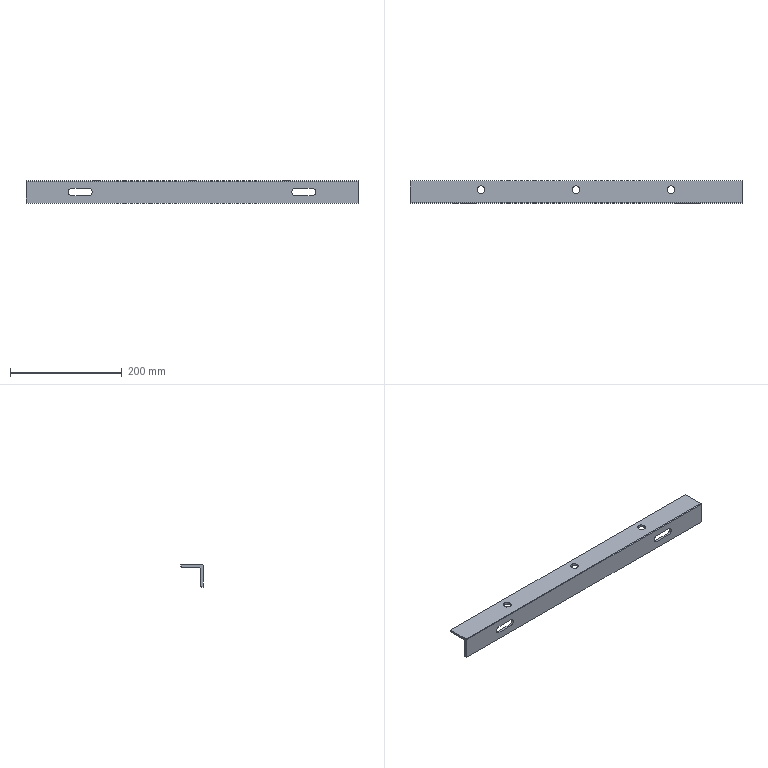Component | SolidWorks | hot-rolled equal angle gb-1 | 1 solid | 26 faces | box 594 x 40 x 40 mm | volume 177153 mm3 | cylinder 14 | plane 12 | commonest cylinder face diameters 14 x6 13 x4 2.667 x2 10 x1 2 x1
build123d program:
from build123d import *

# Parameters (mm, degrees)
BASE_DEPTH          = 594
SKETCH1_2_R         = 7
CUT_EXTRUDE1_DEPTH  = 10
LPATTERN1_COUNT     = 2
LPATTERN1_PITCH     = 170
LPATTERN1_COL_COUNT = 2
LPATTERN1_COL_PITCH = 170
CUT_EXTRUDE2_DEPTH  = 10
FILLET1_R           = 1


with BuildPart() as part:
    # Sketch1 → Base (new body)
    with BuildSketch(Plane.YZ):
        with BuildLine():
            Line((0, 40), (0, 0))
            Line((0, 0), (40, 0))
            Line((40, 0), (40, 2.667))
            ThreePointArc((40, 2.667), (39.609, 3.609), (38.667, 4))
            Line((38.667, 4), (9, 4))
            ThreePointArc((9, 4), (5.464, 5.464), (4, 9))
            Line((4, 9), (4, 38.667))
            ThreePointArc((4, 38.667), (3.609, 39.609), (2.667, 40))
            Line((2.667, 40), (0, 40))
        make_face()
    extrude(amount=BASE_DEPTH)

    # Sketch1_2 → Cut-Extrude1 (cut)
    with BuildSketch(Plane.XY.offset(4)):
        with Locations((297, 24)):
            Circle(SKETCH1_2_R)
    cut_extrude1 = extrude(amount=-CUT_EXTRUDE1_DEPTH, mode=Mode.SUBTRACT)

    # LPattern1: Cut-Extrude1 ×2
    with Locations(*[(-i * LPATTERN1_PITCH, 0, 0) for i in range(1, LPATTERN1_COUNT)]):
        add(cut_extrude1, mode=Mode.SUBTRACT)

    # LPattern1 col: Cut-Extrude1 ×2
    with Locations(*[(i * LPATTERN1_COL_PITCH, 0, 0) for i in range(1, LPATTERN1_COL_COUNT)]):
        add(cut_extrude1, mode=Mode.SUBTRACT)

    # Sketch2 → Cut-Extrude2 (cut)
    with BuildSketch(Plane(origin=(0, 4, 0), x_dir=(1, 0, 0), z_dir=(0, 1, 0))):
        with BuildLine():
            Line((82, -13.5), (112, -13.5))
            ThreePointArc((112, -13.5), (118.5, -20), (112, -26.5))
            Line((112, -26.5), (82, -26.5))
            ThreePointArc((82, -26.5), (75.5, -20), (82, -13.5))
        make_face()
        with BuildLine():
            Line((512, -13.5), (482, -13.5))
            ThreePointArc((482, -13.5), (475.5, -20), (482, -26.5))
            Line((482, -26.5), (512, -26.5))
            ThreePointArc((512, -26.5), (518.5, -20), (512, -13.5))
        make_face()
    extrude(amount=-CUT_EXTRUDE2_DEPTH, mode=Mode.SUBTRACT)

    # Fillet1
    fillet1_edges = [part.edges().sort_by_distance(p)[0] for p in [
        (297, 0, 0),
    ]]
    fillet(fillet1_edges, radius=FILLET1_R)


solid = part.part

# Placed as in the assembly
solid = solid.moved(Location((889.054, 148.5, 997), (-180, 0, 180)))
STEP:
#1=CARTESIAN_POINT('',(16.892,6.791,39.252));
#2=VERTEX_POINT('',#1);
#3=CARTESIAN_POINT('',(16.341,6.791,39.252));
#4=VERTEX_POINT('',#3);
#5=CARTESIAN_POINT('',(16.616,6.791,39.252));
#6=DIRECTION('',(0.,0.,-1.));
#7=DIRECTION('',(-1.,0.,0.));
#8=AXIS2_PLACEMENT_3D('',#5,#6,#7);
#9=CIRCLE('',#8,0.2756);
#10=EDGE_CURVE('',#2,#4,#9,.T.);
#11=ORIENTED_EDGE('',*,*,#10,.F.);
#12=CARTESIAN_POINT('',(16.892,6.791,39.094));
#13=VERTEX_POINT('',#12);
#14=CARTESIAN_POINT('',(16.892,6.791,39.488));
#15=DIRECTION('',(0.,0.,-1.));
#16=VECTOR('',#15,39.37);
#17=LINE('',#14,#16);
#18=EDGE_CURVE('',#2,#13,#17,.T.);
#19=ORIENTED_EDGE('',*,*,#18,.T.);
#20=CARTESIAN_POINT('',(16.341,6.791,39.094));
#21=VERTEX_POINT('',#20);
#22=CARTESIAN_POINT('',(16.616,6.791,39.094));
#23=DIRECTION('',(0.,0.,-1.));
#24=DIRECTION('',(-1.,0.,0.));
#25=AXIS2_PLACEMENT_3D('',#22,#23,#24);
#26=CIRCLE('',#25,0.2756);
#27=EDGE_CURVE('',#13,#21,#26,.T.);
#28=ORIENTED_EDGE('',*,*,#27,.T.);
#29=CARTESIAN_POINT('',(16.341,6.791,39.488));
#30=DIRECTION('',(0.,0.,-1.));
#31=VECTOR('',#30,39.37);
#32=LINE('',#29,#31);
#33=EDGE_CURVE('',#4,#21,#32,.T.);
#34=ORIENTED_EDGE('',*,*,#33,.F.);
#35=EDGE_LOOP('',(#11,#19,#28,#34));
#36=FACE_OUTER_BOUND('',#35,.T.);
#37=CARTESIAN_POINT('',(16.616,6.791,39.488));
#38=DIRECTION('',(0.,0.,-1.));
#39=DIRECTION('',(-1.,0.,0.));
#40=AXIS2_PLACEMENT_3D('',#37,#38,#39);
#41=CYLINDRICAL_SURFACE('',#40,0.2756);
#42=ADVANCED_FACE('',(#36),#41,.F.);
#43=CARTESIAN_POINT('',(30.278,6.791,39.252));
#44=VERTEX_POINT('',#43);
#45=CARTESIAN_POINT('',(29.727,6.791,39.252));
#46=VERTEX_POINT('',#45);
#47=CARTESIAN_POINT('',(30.002,6.791,39.252));
#48=DIRECTION('',(0.,0.,-1.));
#49=DIRECTION('',(-1.,0.,0.));
#50=AXIS2_PLACEMENT_3D('',#47,#48,#49);
#51=CIRCLE('',#50,0.2756);
#52=EDGE_CURVE('',#44,#46,#51,.T.);
#53=ORIENTED_EDGE('',*,*,#52,.F.);
#54=CARTESIAN_POINT('',(30.278,6.791,39.094));
#55=VERTEX_POINT('',#54);
#56=CARTESIAN_POINT('',(30.278,6.791,39.488));
#57=DIRECTION('',(0.,0.,-1.));
#58=VECTOR('',#57,39.37);
#59=LINE('',#56,#58);
#60=EDGE_CURVE('',#44,#55,#59,.T.);
#61=ORIENTED_EDGE('',*,*,#60,.T.);
#62=CARTESIAN_POINT('',(29.727,6.791,39.094));
#63=VERTEX_POINT('',#62);
#64=CARTESIAN_POINT('',(30.002,6.791,39.094));
#65=DIRECTION('',(0.,0.,-1.));
#66=DIRECTION('',(-1.,0.,0.));
#67=AXIS2_PLACEMENT_3D('',#64,#65,#66);
#68=CIRCLE('',#67,0.2756);
#69=EDGE_CURVE('',#55,#63,#68,.T.);
#70=ORIENTED_EDGE('',*,*,#69,.T.);
#71=CARTESIAN_POINT('',(29.727,6.791,39.488));
#72=DIRECTION('',(0.,0.,-1.));
#73=VECTOR('',#72,39.37);
#74=LINE('',#71,#73);
#75=EDGE_CURVE('',#46,#63,#74,.T.);
#76=ORIENTED_EDGE('',*,*,#75,.F.);
#77=EDGE_LOOP('',(#53,#61,#70,#76));
#78=FACE_OUTER_BOUND('',#77,.T.);
#79=CARTESIAN_POINT('',(30.002,6.791,39.488));
#80=DIRECTION('',(0.,0.,-1.));
#81=DIRECTION('',(-1.,0.,0.));
#82=AXIS2_PLACEMENT_3D('',#79,#80,#81);
#83=CYLINDRICAL_SURFACE('',#82,0.2756);
#84=ADVANCED_FACE('',(#78),#83,.F.);
#85=CARTESIAN_POINT('',(23.585,6.791,39.252));
#86=VERTEX_POINT('',#85);
#87=CARTESIAN_POINT('',(23.034,6.791,39.252));
#88=VERTEX_POINT('',#87);
#89=CARTESIAN_POINT('',(23.309,6.791,39.252));
#90=DIRECTION('',(0.,0.,-1.));
#91=DIRECTION('',(-1.,0.,0.));
#92=AXIS2_PLACEMENT_3D('',#89,#90,#91);
#93=CIRCLE('',#92,0.2756);
#94=EDGE_CURVE('',#86,#88,#93,.T.);
#95=ORIENTED_EDGE('',*,*,#94,.F.);
#96=CARTESIAN_POINT('',(23.585,6.791,39.094));
#97=VERTEX_POINT('',#96);
#98=CARTESIAN_POINT('',(23.585,6.791,39.488));
#99=DIRECTION('',(0.,0.,-1.));
#100=VECTOR('',#99,39.37);
#101=LINE('',#98,#100);
#102=EDGE_CURVE('',#86,#97,#101,.T.);
#103=ORIENTED_EDGE('',*,*,#102,.T.);
#104=CARTESIAN_POINT('',(23.034,6.791,39.094));
#105=VERTEX_POINT('',#104);
#106=CARTESIAN_POINT('',(23.309,6.791,39.094));
#107=DIRECTION('',(0.,0.,-1.));
#108=DIRECTION('',(-1.,0.,0.));
#109=AXIS2_PLACEMENT_3D('',#106,#107,#108);
#110=CIRCLE('',#109,0.2756);
#111=EDGE_CURVE('',#97,#105,#110,.T.);
#112=ORIENTED_EDGE('',*,*,#111,.T.);
#113=CARTESIAN_POINT('',(23.034,6.791,39.488));
#114=DIRECTION('',(0.,0.,-1.));
#115=VECTOR('',#114,39.37);
#116=LINE('',#113,#115);
#117=EDGE_CURVE('',#88,#105,#116,.T.);
#118=ORIENTED_EDGE('',*,*,#117,.F.);
#119=EDGE_LOOP('',(#95,#103,#112,#118));
#120=FACE_OUTER_BOUND('',#119,.T.);
#121=CARTESIAN_POINT('',(23.309,6.791,39.488));
#122=DIRECTION('',(0.,0.,-1.));
#123=DIRECTION('',(-1.,0.,0.));
#124=AXIS2_PLACEMENT_3D('',#121,#122,#123);
#125=CYLINDRICAL_SURFACE('',#124,0.2756);
#126=ADVANCED_FACE('',(#120),#125,.F.);
#127=CARTESIAN_POINT('',(35.002,5.951,37.677));
#128=VERTEX_POINT('',#127);
#129=CARTESIAN_POINT('',(35.002,5.846,37.677));
#130=VERTEX_POINT('',#129);
#131=CARTESIAN_POINT('',(35.002,5.846,37.677));
#132=DIRECTION('',(0.,-1.,0.));
#133=VECTOR('',#132,39.37);
#134=LINE('',#131,#133);
#135=EDGE_CURVE('',#128,#130,#134,.T.);
#136=ORIENTED_EDGE('',*,*,#135,.T.);
#137=CARTESIAN_POINT('',(11.616,5.846,37.677));
#138=VERTEX_POINT('',#137);
#139=CARTESIAN_POINT('',(11.616,5.846,37.677));
#140=DIRECTION('',(1.,0.,0.));
#141=VECTOR('',#140,39.37);
#142=LINE('',#139,#141);
#143=EDGE_CURVE('',#138,#130,#142,.T.);
#144=ORIENTED_EDGE('',*,*,#143,.F.);
#145=CARTESIAN_POINT('',(11.616,5.951,37.677));
#146=VERTEX_POINT('',#145);
#147=CARTESIAN_POINT('',(11.616,5.846,37.677));
#148=DIRECTION('',(0.,-1.,0.));
#149=VECTOR('',#148,39.37);
#150=LINE('',#147,#149);
#151=EDGE_CURVE('',#146,#138,#150,.T.);
#152=ORIENTED_EDGE('',*,*,#151,.F.);
#153=CARTESIAN_POINT('',(11.616,5.951,37.677));
#154=DIRECTION('',(1.,0.,0.));
#155=VECTOR('',#154,39.37);
#156=LINE('',#153,#155);
#157=EDGE_CURVE('',#146,#128,#156,.T.);
#158=ORIENTED_EDGE('',*,*,#157,.T.);
#159=EDGE_LOOP('',(#136,#144,#152,#158));
#160=FACE_OUTER_BOUND('',#159,.T.);
#161=CARTESIAN_POINT('',(11.616,5.846,37.677));
#162=DIRECTION('',(0.,0.,1.));
#163=DIRECTION('',(1.,0.,0.));
#164=AXIS2_PLACEMENT_3D('',#161,#162,#163);
#165=PLANE('',#164);
#166=ADVANCED_FACE('',(#160),#165,.F.);
#167=CARTESIAN_POINT('',(16.026,5.846,38.209));
#168=VERTEX_POINT('',#167);
#169=CARTESIAN_POINT('',(14.845,5.846,38.209));
#170=VERTEX_POINT('',#169);
#171=CARTESIAN_POINT('',(11.616,5.846,38.209));
#172=DIRECTION('',(-1.,-0.,-0.));
#173=VECTOR('',#172,39.37);
#174=LINE('',#171,#173);
#175=EDGE_CURVE('',#168,#170,#174,.T.);
#176=ORIENTED_EDGE('',*,*,#175,.T.);
#177=CARTESIAN_POINT('',(14.845,5.846,38.72));
#178=VERTEX_POINT('',#177);
#179=CARTESIAN_POINT('',(14.845,5.846,38.465));
#180=DIRECTION('',(-0.,1.,-0.));
#181=DIRECTION('',(0.,0.,-1.));
#182=AXIS2_PLACEMENT_3D('',#179,#180,#181);
#183=CIRCLE('',#182,0.2559);
#184=EDGE_CURVE('',#170,#178,#183,.T.);
#185=ORIENTED_EDGE('',*,*,#184,.T.);
#186=CARTESIAN_POINT('',(16.026,5.846,38.72));
#187=VERTEX_POINT('',#186);
#188=CARTESIAN_POINT('',(11.616,5.846,38.72));
#189=DIRECTION('',(1.,0.,0.));
#190=VECTOR('',#189,39.37);
#191=LINE('',#188,#190);
#192=EDGE_CURVE('',#178,#187,#191,.T.);
#193=ORIENTED_EDGE('',*,*,#192,.T.);
#194=CARTESIAN_POINT('',(16.026,5.846,38.465));
#195=DIRECTION('',(-0.,1.,-0.));
#196=DIRECTION('',(0.,0.,-1.));
#197=AXIS2_PLACEMENT_3D('',#194,#195,#196);
#198=CIRCLE('',#197,0.2559);
#199=EDGE_CURVE('',#187,#168,#198,.T.);
#200=ORIENTED_EDGE('',*,*,#199,.T.);
#201=EDGE_LOOP('',(#176,#185,#193,#200));
#202=FACE_BOUND('',#201,.T.);
#203=CARTESIAN_POINT('',(30.593,5.846,38.72));
#204=VERTEX_POINT('',#203);
#205=CARTESIAN_POINT('',(31.774,5.846,38.72));
#206=VERTEX_POINT('',#205);
#207=CARTESIAN_POINT('',(11.616,5.846,38.72));
#208=DIRECTION('',(1.,0.,-0.));
#209=VECTOR('',#208,39.37);
#210=LINE('',#207,#209);
#211=EDGE_CURVE('',#204,#206,#210,.T.);
#212=ORIENTED_EDGE('',*,*,#211,.T.);
#213=CARTESIAN_POINT('',(31.774,5.846,38.209));
#214=VERTEX_POINT('',#213);
#215=CARTESIAN_POINT('',(31.774,5.846,38.465));
#216=DIRECTION('',(-0.,1.,-0.));
#217=DIRECTION('',(0.,0.,-1.));
#218=AXIS2_PLACEMENT_3D('',#215,#216,#217);
#219=CIRCLE('',#218,0.2559);
#220=EDGE_CURVE('',#206,#214,#219,.T.);
#221=ORIENTED_EDGE('',*,*,#220,.T.);
#222=CARTESIAN_POINT('',(30.593,5.846,38.209));
#223=VERTEX_POINT('',#222);
#224=CARTESIAN_POINT('',(11.616,5.846,38.209));
#225=DIRECTION('',(-1.,-0.,0.));
#226=VECTOR('',#225,39.37);
#227=LINE('',#224,#226);
#228=EDGE_CURVE('',#214,#223,#227,.T.);
#229=ORIENTED_EDGE('',*,*,#228,.T.);
#230=CARTESIAN_POINT('',(30.593,5.846,38.465));
#231=DIRECTION('',(-0.,1.,-0.));
#232=DIRECTION('',(0.,0.,-1.));
#233=AXIS2_PLACEMENT_3D('',#230,#231,#232);
#234=CIRCLE('',#233,0.2559);
#235=EDGE_CURVE('',#223,#204,#234,.T.);
#236=ORIENTED_EDGE('',*,*,#235,.T.);
#237=EDGE_LOOP('',(#212,#221,#229,#236));
#238=FACE_BOUND('',#237,.T.);
#239=CARTESIAN_POINT('',(35.002,5.846,39.213));
#240=VERTEX_POINT('',#239);
#241=CARTESIAN_POINT('',(35.002,5.846,37.677));
#242=DIRECTION('',(-0.,0.,1.));
#243=VECTOR('',#242,39.37);
#244=LINE('',#241,#243);
#245=EDGE_CURVE('',#130,#240,#244,.T.);
#246=ORIENTED_EDGE('',*,*,#245,.T.);
#247=CARTESIAN_POINT('',(11.616,5.846,39.213));
#248=VERTEX_POINT('',#247);
#249=CARTESIAN_POINT('',(11.616,5.846,39.213));
#250=DIRECTION('',(-1.,-0.,0.));
#251=VECTOR('',#250,39.37);
#252=LINE('',#249,#251);
#253=EDGE_CURVE('',#240,#248,#252,.T.);
#254=ORIENTED_EDGE('',*,*,#253,.T.);
#255=CARTESIAN_POINT('',(11.616,5.846,37.677));
#256=DIRECTION('',(-0.,0.,1.));
#257=VECTOR('',#256,39.37);
#258=LINE('',#255,#257);
#259=EDGE_CURVE('',#138,#248,#258,.T.);
#260=ORIENTED_EDGE('',*,*,#259,.F.);
#261=ORIENTED_EDGE('',*,*,#143,.T.);
#262=EDGE_LOOP('',(#246,#254,#260,#261));
#263=FACE_OUTER_BOUND('',#262,.T.);
#264=CARTESIAN_POINT('',(11.616,5.846,37.677));
#265=DIRECTION('',(-0.,1.,-0.));
#266=DIRECTION('',(0.,-0.,-1.));
#267=AXIS2_PLACEMENT_3D('',#264,#265,#266);
#268=PLANE('',#267);
#269=ADVANCED_FACE('',(#202,#238,#263),#268,.F.);
#270=CARTESIAN_POINT('',(30.002,6.791,39.252));
#271=DIRECTION('',(0.,0.,-1.));
#272=DIRECTION('',(-1.,0.,0.));
#273=AXIS2_PLACEMENT_3D('',#270,#271,#272);
#274=CIRCLE('',#273,0.2756);
#275=EDGE_CURVE('',#46,#44,#274,.T.);
#276=ORIENTED_EDGE('',*,*,#275,.T.);
#277=ORIENTED_EDGE('',*,*,#52,.T.);
#278=EDGE_LOOP('',(#276,#277));
#279=FACE_BOUND('',#278,.T.);
#280=CARTESIAN_POINT('',(23.309,6.791,39.252));
#281=DIRECTION('',(0.,0.,-1.));
#282=DIRECTION('',(-1.,0.,0.));
#283=AXIS2_PLACEMENT_3D('',#280,#281,#282);
#284=CIRCLE('',#283,0.2756);
#285=EDGE_CURVE('',#88,#86,#284,.T.);
#286=ORIENTED_EDGE('',*,*,#285,.T.);
#287=ORIENTED_EDGE('',*,*,#94,.T.);
#288=EDGE_LOOP('',(#286,#287));
#289=FACE_BOUND('',#288,.T.);
#290=CARTESIAN_POINT('',(11.616,5.886,39.252));
#291=VERTEX_POINT('',#290);
#292=CARTESIAN_POINT('',(11.616,7.421,39.252));
#293=VERTEX_POINT('',#292);
#294=CARTESIAN_POINT('',(11.616,5.846,39.252));
#295=DIRECTION('',(-0.,1.,0.));
#296=VECTOR('',#295,39.37);
#297=LINE('',#294,#296);
#298=EDGE_CURVE('',#291,#293,#297,.T.);
#299=ORIENTED_EDGE('',*,*,#298,.F.);
#300=CARTESIAN_POINT('',(35.002,5.886,39.252));
#301=VERTEX_POINT('',#300);
#302=CARTESIAN_POINT('',(11.616,5.886,39.252));
#303=DIRECTION('',(1.,0.,0.));
#304=VECTOR('',#303,39.37);
#305=LINE('',#302,#304);
#306=EDGE_CURVE('',#291,#301,#305,.T.);
#307=ORIENTED_EDGE('',*,*,#306,.T.);
#308=CARTESIAN_POINT('',(35.002,7.421,39.252));
#309=VERTEX_POINT('',#308);
#310=CARTESIAN_POINT('',(35.002,5.846,39.252));
#311=DIRECTION('',(-0.,1.,0.));
#312=VECTOR('',#311,39.37);
#313=LINE('',#310,#312);
#314=EDGE_CURVE('',#301,#309,#313,.T.);
#315=ORIENTED_EDGE('',*,*,#314,.T.);
#316=CARTESIAN_POINT('',(11.616,7.421,39.252));
#317=DIRECTION('',(1.,0.,0.));
#318=VECTOR('',#317,39.37);
#319=LINE('',#316,#318);
#320=EDGE_CURVE('',#293,#309,#319,.T.);
#321=ORIENTED_EDGE('',*,*,#320,.F.);
#322=EDGE_LOOP('',(#299,#307,#315,#321));
#323=FACE_OUTER_BOUND('',#322,.T.);
#324=CARTESIAN_POINT('',(16.616,6.791,39.252));
#325=DIRECTION('',(0.,0.,-1.));
#326=DIRECTION('',(-1.,0.,0.));
#327=AXIS2_PLACEMENT_3D('',#324,#325,#326);
#328=CIRCLE('',#327,0.2756);
#329=EDGE_CURVE('',#4,#2,#328,.T.);
#330=ORIENTED_EDGE('',*,*,#329,.T.);
#331=ORIENTED_EDGE('',*,*,#10,.T.);
#332=EDGE_LOOP('',(#330,#331));
#333=FACE_BOUND('',#332,.T.);
#334=CARTESIAN_POINT('',(11.616,5.846,39.252));
#335=DIRECTION('',(0.,0.,-1.));
#336=DIRECTION('',(-1.,-0.,0.));
#337=AXIS2_PLACEMENT_3D('',#334,#335,#336);
#338=PLANE('',#337);
#339=ADVANCED_FACE('',(#279,#289,#323,#333),#338,.F.);
#340=CARTESIAN_POINT('',(35.002,7.421,39.147));
#341=VERTEX_POINT('',#340);
#342=CARTESIAN_POINT('',(35.002,7.421,39.252));
#343=DIRECTION('',(0.,0.,-1.));
#344=VECTOR('',#343,39.37);
#345=LINE('',#342,#344);
#346=EDGE_CURVE('',#309,#341,#345,.T.);
#347=ORIENTED_EDGE('',*,*,#346,.T.);
#348=CARTESIAN_POINT('',(11.616,7.421,39.147));
#349=VERTEX_POINT('',#348);
#350=CARTESIAN_POINT('',(11.616,7.421,39.147));
#351=DIRECTION('',(1.,0.,0.));
#352=VECTOR('',#351,39.37);
#353=LINE('',#350,#352);
#354=EDGE_CURVE('',#349,#341,#353,.T.);
#355=ORIENTED_EDGE('',*,*,#354,.F.);
#356=CARTESIAN_POINT('',(11.616,7.421,39.252));
#357=DIRECTION('',(0.,0.,-1.));
#358=VECTOR('',#357,39.37);
#359=LINE('',#356,#358);
#360=EDGE_CURVE('',#293,#349,#359,.T.);
#361=ORIENTED_EDGE('',*,*,#360,.F.);
#362=ORIENTED_EDGE('',*,*,#320,.T.);
#363=EDGE_LOOP('',(#347,#355,#361,#362));
#364=FACE_OUTER_BOUND('',#363,.T.);
#365=CARTESIAN_POINT('',(11.616,7.421,39.252));
#366=DIRECTION('',(0.,-1.,0.));
#367=DIRECTION('',(0.,0.,1.));
#368=AXIS2_PLACEMENT_3D('',#365,#366,#367);
#369=PLANE('',#368);
#370=ADVANCED_FACE('',(#364),#369,.F.);
#371=CARTESIAN_POINT('',(35.002,7.369,39.094));
#372=VERTEX_POINT('',#371);
#373=CARTESIAN_POINT('',(35.002,7.369,39.147));
#374=DIRECTION('',(-1.,-0.,0.));
#375=DIRECTION('',(0.,0.,1.));
#376=AXIS2_PLACEMENT_3D('',#373,#374,#375);
#377=CIRCLE('',#376,0.05249);
#378=EDGE_CURVE('',#341,#372,#377,.T.);
#379=ORIENTED_EDGE('',*,*,#378,.T.);
#380=CARTESIAN_POINT('',(11.616,7.369,39.094));
#381=VERTEX_POINT('',#380);
#382=CARTESIAN_POINT('',(11.616,7.369,39.094));
#383=DIRECTION('',(1.,0.,0.));
#384=VECTOR('',#383,39.37);
#385=LINE('',#382,#384);
#386=EDGE_CURVE('',#381,#372,#385,.T.);
#387=ORIENTED_EDGE('',*,*,#386,.F.);
#388=CARTESIAN_POINT('',(11.616,7.369,39.147));
#389=DIRECTION('',(-1.,-0.,0.));
#390=DIRECTION('',(0.,0.,1.));
#391=AXIS2_PLACEMENT_3D('',#388,#389,#390);
#392=CIRCLE('',#391,0.05249);
#393=EDGE_CURVE('',#349,#381,#392,.T.);
#394=ORIENTED_EDGE('',*,*,#393,.F.);
#395=ORIENTED_EDGE('',*,*,#354,.T.);
#396=EDGE_LOOP('',(#379,#387,#394,#395));
#397=FACE_OUTER_BOUND('',#396,.T.);
#398=CARTESIAN_POINT('',(11.616,7.369,39.147));
#399=DIRECTION('',(1.,0.,0.));
#400=DIRECTION('',(0.,0.,-1.));
#401=AXIS2_PLACEMENT_3D('',#398,#399,#400);
#402=CYLINDRICAL_SURFACE('',#401,0.05249);
#403=ADVANCED_FACE('',(#397),#402,.T.);
#404=CARTESIAN_POINT('',(30.002,6.791,39.094));
#405=DIRECTION('',(0.,0.,-1.));
#406=DIRECTION('',(-1.,0.,0.));
#407=AXIS2_PLACEMENT_3D('',#404,#405,#406);
#408=CIRCLE('',#407,0.2756);
#409=EDGE_CURVE('',#63,#55,#408,.T.);
#410=ORIENTED_EDGE('',*,*,#409,.F.);
#411=ORIENTED_EDGE('',*,*,#69,.F.);
#412=EDGE_LOOP('',(#410,#411));
#413=FACE_BOUND('',#412,.T.);
#414=CARTESIAN_POINT('',(23.309,6.791,39.094));
#415=DIRECTION('',(0.,0.,-1.));
#416=DIRECTION('',(-1.,0.,0.));
#417=AXIS2_PLACEMENT_3D('',#414,#415,#416);
#418=CIRCLE('',#417,0.2756);
#419=EDGE_CURVE('',#105,#97,#418,.T.);
#420=ORIENTED_EDGE('',*,*,#419,.F.);
#421=ORIENTED_EDGE('',*,*,#111,.F.);
#422=EDGE_LOOP('',(#420,#421));
#423=FACE_BOUND('',#422,.T.);
#424=CARTESIAN_POINT('',(35.002,6.201,39.094));
#425=VERTEX_POINT('',#424);
#426=CARTESIAN_POINT('',(35.002,6.201,39.094));
#427=DIRECTION('',(0.,-1.,0.));
#428=VECTOR('',#427,39.37);
#429=LINE('',#426,#428);
#430=EDGE_CURVE('',#372,#425,#429,.T.);
#431=ORIENTED_EDGE('',*,*,#430,.T.);
#432=CARTESIAN_POINT('',(11.616,6.201,39.094));
#433=VERTEX_POINT('',#432);
#434=CARTESIAN_POINT('',(11.616,6.201,39.094));
#435=DIRECTION('',(1.,0.,0.));
#436=VECTOR('',#435,39.37);
#437=LINE('',#434,#436);
#438=EDGE_CURVE('',#433,#425,#437,.T.);
#439=ORIENTED_EDGE('',*,*,#438,.F.);
#440=CARTESIAN_POINT('',(11.616,6.201,39.094));
#441=DIRECTION('',(0.,-1.,0.));
#442=VECTOR('',#441,39.37);
#443=LINE('',#440,#442);
#444=EDGE_CURVE('',#381,#433,#443,.T.);
#445=ORIENTED_EDGE('',*,*,#444,.F.);
#446=ORIENTED_EDGE('',*,*,#386,.T.);
#447=EDGE_LOOP('',(#431,#439,#445,#446));
#448=FACE_OUTER_BOUND('',#447,.T.);
#449=CARTESIAN_POINT('',(16.616,6.791,39.094));
#450=DIRECTION('',(0.,0.,-1.));
#451=DIRECTION('',(-1.,0.,0.));
#452=AXIS2_PLACEMENT_3D('',#449,#450,#451);
#453=CIRCLE('',#452,0.2756);
#454=EDGE_CURVE('',#21,#13,#453,.T.);
#455=ORIENTED_EDGE('',*,*,#454,.F.);
#456=ORIENTED_EDGE('',*,*,#27,.F.);
#457=EDGE_LOOP('',(#455,#456));
#458=FACE_BOUND('',#457,.T.);
#459=CARTESIAN_POINT('',(11.616,6.201,39.094));
#460=DIRECTION('',(-0.,0.,1.));
#461=DIRECTION('',(-0.,1.,-0.));
#462=AXIS2_PLACEMENT_3D('',#459,#460,#461);
#463=PLANE('',#462);
#464=ADVANCED_FACE('',(#413,#423,#448,#458),#463,.F.);
#465=CARTESIAN_POINT('',(35.002,6.004,38.898));
#466=VERTEX_POINT('',#465);
#467=CARTESIAN_POINT('',(35.002,6.201,38.898));
#468=DIRECTION('',(1.,0.,0.));
#469=DIRECTION('',(0.,0.,1.));
#470=AXIS2_PLACEMENT_3D('',#467,#468,#469);
#471=CIRCLE('',#470,0.1969);
#472=EDGE_CURVE('',#425,#466,#471,.T.);
#473=ORIENTED_EDGE('',*,*,#472,.T.);
#474=CARTESIAN_POINT('',(11.616,6.004,38.898));
#475=VERTEX_POINT('',#474);
#476=CARTESIAN_POINT('',(11.616,6.004,38.898));
#477=DIRECTION('',(1.,0.,0.));
#478=VECTOR('',#477,39.37);
#479=LINE('',#476,#478);
#480=EDGE_CURVE('',#475,#466,#479,.T.);
#481=ORIENTED_EDGE('',*,*,#480,.F.);
#482=CARTESIAN_POINT('',(11.616,6.201,38.898));
#483=DIRECTION('',(1.,0.,0.));
#484=DIRECTION('',(0.,0.,1.));
#485=AXIS2_PLACEMENT_3D('',#482,#483,#484);
#486=CIRCLE('',#485,0.1969);
#487=EDGE_CURVE('',#433,#475,#486,.T.);
#488=ORIENTED_EDGE('',*,*,#487,.F.);
#489=ORIENTED_EDGE('',*,*,#438,.T.);
#490=EDGE_LOOP('',(#473,#481,#488,#489));
#491=FACE_OUTER_BOUND('',#490,.T.);
#492=CARTESIAN_POINT('',(11.616,6.201,38.898));
#493=DIRECTION('',(1.,0.,0.));
#494=DIRECTION('',(0.,0.,-1.));
#495=AXIS2_PLACEMENT_3D('',#492,#493,#494);
#496=CYLINDRICAL_SURFACE('',#495,0.1969);
#497=ADVANCED_FACE('',(#491),#496,.F.);
#498=CARTESIAN_POINT('',(14.845,6.004,38.72));
#499=VERTEX_POINT('',#498);
#500=CARTESIAN_POINT('',(16.026,6.004,38.72));
#501=VERTEX_POINT('',#500);
#502=CARTESIAN_POINT('',(14.845,6.004,38.72));
#503=DIRECTION('',(1.,0.,0.));
#504=VECTOR('',#503,39.37);
#505=LINE('',#502,#504);
#506=EDGE_CURVE('',#499,#501,#505,.T.);
#507=ORIENTED_EDGE('',*,*,#506,.F.);
#508=CARTESIAN_POINT('',(14.845,6.004,38.209));
#509=VERTEX_POINT('',#508);
#510=CARTESIAN_POINT('',(14.845,6.004,38.465));
#511=DIRECTION('',(-0.,1.,-0.));
#512=DIRECTION('',(0.,0.,1.));
#513=AXIS2_PLACEMENT_3D('',#510,#511,#512);
#514=CIRCLE('',#513,0.2559);
#515=EDGE_CURVE('',#509,#499,#514,.T.);
#516=ORIENTED_EDGE('',*,*,#515,.F.);
#517=CARTESIAN_POINT('',(16.026,6.004,38.209));
#518=VERTEX_POINT('',#517);
#519=CARTESIAN_POINT('',(14.845,6.004,38.209));
#520=DIRECTION('',(-1.,-0.,-0.));
#521=VECTOR('',#520,39.37);
#522=LINE('',#519,#521);
#523=EDGE_CURVE('',#518,#509,#522,.T.);
#524=ORIENTED_EDGE('',*,*,#523,.F.);
#525=CARTESIAN_POINT('',(16.026,6.004,38.465));
#526=DIRECTION('',(-0.,1.,-0.));
#527=DIRECTION('',(0.,0.,1.));
#528=AXIS2_PLACEMENT_3D('',#525,#526,#527);
#529=CIRCLE('',#528,0.2559);
#530=EDGE_CURVE('',#501,#518,#529,.T.);
#531=ORIENTED_EDGE('',*,*,#530,.F.);
#532=EDGE_LOOP('',(#507,#516,#524,#531));
#533=FACE_BOUND('',#532,.T.);
#534=CARTESIAN_POINT('',(31.774,6.004,38.209));
#535=VERTEX_POINT('',#534);
#536=CARTESIAN_POINT('',(30.593,6.004,38.209));
#537=VERTEX_POINT('',#536);
#538=CARTESIAN_POINT('',(31.774,6.004,38.209));
#539=DIRECTION('',(-1.,-0.,0.));
#540=VECTOR('',#539,39.37);
#541=LINE('',#538,#540);
#542=EDGE_CURVE('',#535,#537,#541,.T.);
#543=ORIENTED_EDGE('',*,*,#542,.F.);
#544=CARTESIAN_POINT('',(31.774,6.004,38.72));
#545=VERTEX_POINT('',#544);
#546=CARTESIAN_POINT('',(31.774,6.004,38.465));
#547=DIRECTION('',(-0.,1.,-0.));
#548=DIRECTION('',(0.,0.,-1.));
#549=AXIS2_PLACEMENT_3D('',#546,#547,#548);
#550=CIRCLE('',#549,0.2559);
#551=EDGE_CURVE('',#545,#535,#550,.T.);
#552=ORIENTED_EDGE('',*,*,#551,.F.);
#553=CARTESIAN_POINT('',(30.593,6.004,38.72));
#554=VERTEX_POINT('',#553);
#555=CARTESIAN_POINT('',(31.774,6.004,38.72));
#556=DIRECTION('',(1.,0.,-0.));
#557=VECTOR('',#556,39.37);
#558=LINE('',#555,#557);
#559=EDGE_CURVE('',#554,#545,#558,.T.);
#560=ORIENTED_EDGE('',*,*,#559,.F.);
#561=CARTESIAN_POINT('',(30.593,6.004,38.465));
#562=DIRECTION('',(-0.,1.,-0.));
#563=DIRECTION('',(0.,0.,-1.));
#564=AXIS2_PLACEMENT_3D('',#561,#562,#563);
#565=CIRCLE('',#564,0.2559);
#566=EDGE_CURVE('',#537,#554,#565,.T.);
#567=ORIENTED_EDGE('',*,*,#566,.F.);
#568=EDGE_LOOP('',(#543,#552,#560,#567));
#569=FACE_BOUND('',#568,.T.);
#570=CARTESIAN_POINT('',(35.002,6.004,37.73));
#571=VERTEX_POINT('',#570);
#572=CARTESIAN_POINT('',(35.002,6.004,37.73));
#573=DIRECTION('',(0.,-0.,-1.));
#574=VECTOR('',#573,39.37);
#575=LINE('',#572,#574);
#576=EDGE_CURVE('',#466,#571,#575,.T.);
#577=ORIENTED_EDGE('',*,*,#576,.T.);
#578=CARTESIAN_POINT('',(11.616,6.004,37.73));
#579=VERTEX_POINT('',#578);
#580=CARTESIAN_POINT('',(11.616,6.004,37.73));
#581=DIRECTION('',(1.,0.,0.));
#582=VECTOR('',#581,39.37);
#583=LINE('',#580,#582);
#584=EDGE_CURVE('',#579,#571,#583,.T.);
#585=ORIENTED_EDGE('',*,*,#584,.F.);
#586=CARTESIAN_POINT('',(11.616,6.004,37.73));
#587=DIRECTION('',(0.,-0.,-1.));
#588=VECTOR('',#587,39.37);
#589=LINE('',#586,#588);
#590=EDGE_CURVE('',#475,#579,#589,.T.);
#591=ORIENTED_EDGE('',*,*,#590,.F.);
#592=ORIENTED_EDGE('',*,*,#480,.T.);
#593=EDGE_LOOP('',(#577,#585,#591,#592));
#594=FACE_OUTER_BOUND('',#593,.T.);
#595=CARTESIAN_POINT('',(11.616,6.004,37.73));
#596=DIRECTION('',(0.,-1.,0.));
#597=DIRECTION('',(-0.,0.,1.));
#598=AXIS2_PLACEMENT_3D('',#595,#596,#597);
#599=PLANE('',#598);
#600=ADVANCED_FACE('',(#533,#569,#594),#599,.F.);
#601=CARTESIAN_POINT('',(35.002,5.951,37.73));
#602=DIRECTION('',(-1.,-0.,0.));
#603=DIRECTION('',(0.,0.,-1.));
#604=AXIS2_PLACEMENT_3D('',#601,#602,#603);
#605=CIRCLE('',#604,0.05249);
#606=EDGE_CURVE('',#571,#128,#605,.T.);
#607=ORIENTED_EDGE('',*,*,#606,.T.);
#608=ORIENTED_EDGE('',*,*,#157,.F.);
#609=CARTESIAN_POINT('',(11.616,5.951,37.73));
#610=DIRECTION('',(-1.,-0.,0.));
#611=DIRECTION('',(0.,0.,-1.));
#612=AXIS2_PLACEMENT_3D('',#609,#610,#611);
#613=CIRCLE('',#612,0.05249);
#614=EDGE_CURVE('',#579,#146,#613,.T.);
#615=ORIENTED_EDGE('',*,*,#614,.F.);
#616=ORIENTED_EDGE('',*,*,#584,.T.);
#617=EDGE_LOOP('',(#607,#608,#615,#616));
#618=FACE_OUTER_BOUND('',#617,.T.);
#619=CARTESIAN_POINT('',(11.616,5.951,37.73));
#620=DIRECTION('',(1.,0.,0.));
#621=DIRECTION('',(0.,0.,-1.));
#622=AXIS2_PLACEMENT_3D('',#619,#620,#621);
#623=CYLINDRICAL_SURFACE('',#622,0.05249);
#624=ADVANCED_FACE('',(#618),#623,.T.);
#625=ORIENTED_EDGE('',*,*,#259,.T.);
#626=CARTESIAN_POINT('',(11.616,5.886,39.213));
#627=DIRECTION('',(-1.,-0.,0.));
#628=DIRECTION('',(0.,0.,-1.));
#629=AXIS2_PLACEMENT_3D('',#626,#627,#628);
#630=CIRCLE('',#629,0.03937);
#631=EDGE_CURVE('',#248,#291,#630,.T.);
#632=ORIENTED_EDGE('',*,*,#631,.T.);
#633=ORIENTED_EDGE('',*,*,#298,.T.);
#634=ORIENTED_EDGE('',*,*,#360,.T.);
#635=ORIENTED_EDGE('',*,*,#393,.T.);
#636=ORIENTED_EDGE('',*,*,#444,.T.);
#637=ORIENTED_EDGE('',*,*,#487,.T.);
#638=ORIENTED_EDGE('',*,*,#590,.T.);
#639=ORIENTED_EDGE('',*,*,#614,.T.);
#640=ORIENTED_EDGE('',*,*,#151,.T.);
#641=EDGE_LOOP('',(#625,#632,#633,#634,#635,#636,#637,#638,#639,#640));
#642=FACE_OUTER_BOUND('',#641,.T.);
#643=CARTESIAN_POINT('',(11.616,5.951,37.73));
#644=DIRECTION('',(1.,0.,0.));
#645=DIRECTION('',(0.,0.,-1.));
#646=AXIS2_PLACEMENT_3D('',#643,#644,#645);
#647=PLANE('',#646);
#648=ADVANCED_FACE('',(#642),#647,.F.);
#649=ORIENTED_EDGE('',*,*,#314,.F.);
#650=CARTESIAN_POINT('',(35.002,5.886,39.213));
#651=DIRECTION('',(1.,0.,0.));
#652=DIRECTION('',(0.,0.,-1.));
#653=AXIS2_PLACEMENT_3D('',#650,#651,#652);
#654=CIRCLE('',#653,0.03937);
#655=EDGE_CURVE('',#301,#240,#654,.T.);
#656=ORIENTED_EDGE('',*,*,#655,.T.);
#657=ORIENTED_EDGE('',*,*,#245,.F.);
#658=ORIENTED_EDGE('',*,*,#135,.F.);
#659=ORIENTED_EDGE('',*,*,#606,.F.);
#660=ORIENTED_EDGE('',*,*,#576,.F.);
#661=ORIENTED_EDGE('',*,*,#472,.F.);
#662=ORIENTED_EDGE('',*,*,#430,.F.);
#663=ORIENTED_EDGE('',*,*,#378,.F.);
#664=ORIENTED_EDGE('',*,*,#346,.F.);
#665=EDGE_LOOP('',(#649,#656,#657,#658,#659,#660,#661,#662,#663,#664));
#666=FACE_OUTER_BOUND('',#665,.T.);
#667=CARTESIAN_POINT('',(35.002,5.951,37.73));
#668=DIRECTION('',(1.,0.,0.));
#669=DIRECTION('',(0.,0.,-1.));
#670=AXIS2_PLACEMENT_3D('',#667,#668,#669);
#671=PLANE('',#670);
#672=ADVANCED_FACE('',(#666),#671,.T.);
#673=ORIENTED_EDGE('',*,*,#102,.F.);
#674=ORIENTED_EDGE('',*,*,#285,.F.);
#675=ORIENTED_EDGE('',*,*,#117,.T.);
#676=ORIENTED_EDGE('',*,*,#419,.T.);
#677=EDGE_LOOP('',(#673,#674,#675,#676));
#678=FACE_OUTER_BOUND('',#677,.T.);
#679=CARTESIAN_POINT('',(23.309,6.791,39.488));
#680=DIRECTION('',(0.,0.,-1.));
#681=DIRECTION('',(-1.,0.,0.));
#682=AXIS2_PLACEMENT_3D('',#679,#680,#681);
#683=CYLINDRICAL_SURFACE('',#682,0.2756);
#684=ADVANCED_FACE('',(#678),#683,.F.);
#685=ORIENTED_EDGE('',*,*,#60,.F.);
#686=ORIENTED_EDGE('',*,*,#275,.F.);
#687=ORIENTED_EDGE('',*,*,#75,.T.);
#688=ORIENTED_EDGE('',*,*,#409,.T.);
#689=EDGE_LOOP('',(#685,#686,#687,#688));
#690=FACE_OUTER_BOUND('',#689,.T.);
#691=CARTESIAN_POINT('',(30.002,6.791,39.488));
#692=DIRECTION('',(0.,0.,-1.));
#693=DIRECTION('',(-1.,0.,0.));
#694=AXIS2_PLACEMENT_3D('',#691,#692,#693);
#695=CYLINDRICAL_SURFACE('',#694,0.2756);
#696=ADVANCED_FACE('',(#690),#695,.F.);
#697=ORIENTED_EDGE('',*,*,#18,.F.);
#698=ORIENTED_EDGE('',*,*,#329,.F.);
#699=ORIENTED_EDGE('',*,*,#33,.T.);
#700=ORIENTED_EDGE('',*,*,#454,.T.);
#701=EDGE_LOOP('',(#697,#698,#699,#700));
#702=FACE_OUTER_BOUND('',#701,.T.);
#703=CARTESIAN_POINT('',(16.616,6.791,39.488));
#704=DIRECTION('',(0.,0.,-1.));
#705=DIRECTION('',(-1.,0.,0.));
#706=AXIS2_PLACEMENT_3D('',#703,#704,#705);
#707=CYLINDRICAL_SURFACE('',#706,0.2756);
#708=ADVANCED_FACE('',(#702),#707,.F.);
#709=CARTESIAN_POINT('',(31.774,5.61,38.72));
#710=DIRECTION('',(-0.,1.,-0.));
#711=VECTOR('',#710,39.37);
#712=LINE('',#709,#711);
#713=EDGE_CURVE('',#206,#545,#712,.T.);
#714=ORIENTED_EDGE('',*,*,#713,.T.);
#715=ORIENTED_EDGE('',*,*,#551,.T.);
#716=CARTESIAN_POINT('',(31.774,5.61,38.209));
#717=DIRECTION('',(-0.,1.,-0.));
#718=VECTOR('',#717,39.37);
#719=LINE('',#716,#718);
#720=EDGE_CURVE('',#214,#535,#719,.T.);
#721=ORIENTED_EDGE('',*,*,#720,.F.);
#722=ORIENTED_EDGE('',*,*,#220,.F.);
#723=EDGE_LOOP('',(#714,#715,#721,#722));
#724=FACE_OUTER_BOUND('',#723,.T.);
#725=CARTESIAN_POINT('',(31.774,5.61,38.465));
#726=DIRECTION('',(-0.,1.,-0.));
#727=DIRECTION('',(0.,0.,-1.));
#728=AXIS2_PLACEMENT_3D('',#725,#726,#727);
#729=CYLINDRICAL_SURFACE('',#728,0.2559);
#730=ADVANCED_FACE('',(#724),#729,.F.);
#731=CARTESIAN_POINT('',(30.593,5.61,38.72));
#732=DIRECTION('',(-0.,1.,-0.));
#733=VECTOR('',#732,39.37);
#734=LINE('',#731,#733);
#735=EDGE_CURVE('',#204,#554,#734,.T.);
#736=ORIENTED_EDGE('',*,*,#735,.T.);
#737=ORIENTED_EDGE('',*,*,#559,.T.);
#738=ORIENTED_EDGE('',*,*,#713,.F.);
#739=ORIENTED_EDGE('',*,*,#211,.F.);
#740=EDGE_LOOP('',(#736,#737,#738,#739));
#741=FACE_OUTER_BOUND('',#740,.T.);
#742=CARTESIAN_POINT('',(31.774,5.61,38.72));
#743=DIRECTION('',(0.,0.,1.));
#744=DIRECTION('',(1.,0.,-0.));
#745=AXIS2_PLACEMENT_3D('',#742,#743,#744);
#746=PLANE('',#745);
#747=ADVANCED_FACE('',(#741),#746,.F.);
#748=CARTESIAN_POINT('',(30.593,5.61,38.209));
#749=DIRECTION('',(-0.,1.,-0.));
#750=VECTOR('',#749,39.37);
#751=LINE('',#748,#750);
#752=EDGE_CURVE('',#223,#537,#751,.T.);
#753=ORIENTED_EDGE('',*,*,#752,.T.);
#754=ORIENTED_EDGE('',*,*,#566,.T.);
#755=ORIENTED_EDGE('',*,*,#735,.F.);
#756=ORIENTED_EDGE('',*,*,#235,.F.);
#757=EDGE_LOOP('',(#753,#754,#755,#756));
#758=FACE_OUTER_BOUND('',#757,.T.);
#759=CARTESIAN_POINT('',(30.593,5.61,38.465));
#760=DIRECTION('',(-0.,1.,-0.));
#761=DIRECTION('',(0.,0.,-1.));
#762=AXIS2_PLACEMENT_3D('',#759,#760,#761);
#763=CYLINDRICAL_SURFACE('',#762,0.2559);
#764=ADVANCED_FACE('',(#758),#763,.F.);
#765=ORIENTED_EDGE('',*,*,#720,.T.);
#766=ORIENTED_EDGE('',*,*,#542,.T.);
#767=ORIENTED_EDGE('',*,*,#752,.F.);
#768=ORIENTED_EDGE('',*,*,#228,.F.);
#769=EDGE_LOOP('',(#765,#766,#767,#768));
#770=FACE_OUTER_BOUND('',#769,.T.);
#771=CARTESIAN_POINT('',(31.774,5.61,38.209));
#772=DIRECTION('',(-0.,-0.,-1.));
#773=DIRECTION('',(-1.,-0.,0.));
#774=AXIS2_PLACEMENT_3D('',#771,#772,#773);
#775=PLANE('',#774);
#776=ADVANCED_FACE('',(#770),#775,.F.);
#777=CARTESIAN_POINT('',(14.845,5.61,38.209));
#778=DIRECTION('',(-0.,1.,-0.));
#779=VECTOR('',#778,39.37);
#780=LINE('',#777,#779);
#781=EDGE_CURVE('',#170,#509,#780,.T.);
#782=ORIENTED_EDGE('',*,*,#781,.T.);
#783=ORIENTED_EDGE('',*,*,#515,.T.);
#784=CARTESIAN_POINT('',(14.845,5.61,38.72));
#785=DIRECTION('',(-0.,1.,-0.));
#786=VECTOR('',#785,39.37);
#787=LINE('',#784,#786);
#788=EDGE_CURVE('',#178,#499,#787,.T.);
#789=ORIENTED_EDGE('',*,*,#788,.F.);
#790=ORIENTED_EDGE('',*,*,#184,.F.);
#791=EDGE_LOOP('',(#782,#783,#789,#790));
#792=FACE_OUTER_BOUND('',#791,.T.);
#793=CARTESIAN_POINT('',(14.845,5.61,38.465));
#794=DIRECTION('',(-0.,1.,-0.));
#795=DIRECTION('',(0.,0.,-1.));
#796=AXIS2_PLACEMENT_3D('',#793,#794,#795);
#797=CYLINDRICAL_SURFACE('',#796,0.2559);
#798=ADVANCED_FACE('',(#792),#797,.F.);
#799=CARTESIAN_POINT('',(16.026,5.61,38.209));
#800=DIRECTION('',(-0.,1.,-0.));
#801=VECTOR('',#800,39.37);
#802=LINE('',#799,#801);
#803=EDGE_CURVE('',#168,#518,#802,.T.);
#804=ORIENTED_EDGE('',*,*,#803,.T.);
#805=ORIENTED_EDGE('',*,*,#523,.T.);
#806=ORIENTED_EDGE('',*,*,#781,.F.);
#807=ORIENTED_EDGE('',*,*,#175,.F.);
#808=EDGE_LOOP('',(#804,#805,#806,#807));
#809=FACE_OUTER_BOUND('',#808,.T.);
#810=CARTESIAN_POINT('',(14.845,5.61,38.209));
#811=DIRECTION('',(0.,-0.,-1.));
#812=DIRECTION('',(-1.,-0.,-0.));
#813=AXIS2_PLACEMENT_3D('',#810,#811,#812);
#814=PLANE('',#813);
#815=ADVANCED_FACE('',(#809),#814,.F.);
#816=CARTESIAN_POINT('',(16.026,5.61,38.72));
#817=DIRECTION('',(-0.,1.,-0.));
#818=VECTOR('',#817,39.37);
#819=LINE('',#816,#818);
#820=EDGE_CURVE('',#187,#501,#819,.T.);
#821=ORIENTED_EDGE('',*,*,#820,.T.);
#822=ORIENTED_EDGE('',*,*,#530,.T.);
#823=ORIENTED_EDGE('',*,*,#803,.F.);
#824=ORIENTED_EDGE('',*,*,#199,.F.);
#825=EDGE_LOOP('',(#821,#822,#823,#824));
#826=FACE_OUTER_BOUND('',#825,.T.);
#827=CARTESIAN_POINT('',(16.026,5.61,38.465));
#828=DIRECTION('',(-0.,1.,-0.));
#829=DIRECTION('',(0.,0.,-1.));
#830=AXIS2_PLACEMENT_3D('',#827,#828,#829);
#831=CYLINDRICAL_SURFACE('',#830,0.2559);
#832=ADVANCED_FACE('',(#826),#831,.F.);
#833=ORIENTED_EDGE('',*,*,#788,.T.);
#834=ORIENTED_EDGE('',*,*,#506,.T.);
#835=ORIENTED_EDGE('',*,*,#820,.F.);
#836=ORIENTED_EDGE('',*,*,#192,.F.);
#837=EDGE_LOOP('',(#833,#834,#835,#836));
#838=FACE_OUTER_BOUND('',#837,.T.);
#839=CARTESIAN_POINT('',(14.845,5.61,38.72));
#840=DIRECTION('',(-0.,0.,1.));
#841=DIRECTION('',(1.,0.,0.));
#842=AXIS2_PLACEMENT_3D('',#839,#840,#841);
#843=PLANE('',#842);
#844=ADVANCED_FACE('',(#838),#843,.F.);
#845=ORIENTED_EDGE('',*,*,#631,.F.);
#846=ORIENTED_EDGE('',*,*,#253,.F.);
#847=ORIENTED_EDGE('',*,*,#655,.F.);
#848=ORIENTED_EDGE('',*,*,#306,.F.);
#849=EDGE_LOOP('',(#845,#846,#847,#848));
#850=FACE_OUTER_BOUND('',#849,.T.);
#851=CARTESIAN_POINT('',(11.616,5.886,39.213));
#852=DIRECTION('',(1.,0.,0.));
#853=DIRECTION('',(0.,0.,-1.));
#854=AXIS2_PLACEMENT_3D('',#851,#852,#853);
#855=CYLINDRICAL_SURFACE('',#854,0.03937);
#856=ADVANCED_FACE('',(#850),#855,.T.);
#857=CLOSED_SHELL('',(#42,#84,#126,#166,#269,#339,#370,#403,#464,#497,#600,#624,#648,#672,#684,#696,#708,#730,#747,#764,#776,#798,#815,#832,#844,#856));
#858=MANIFOLD_SOLID_BREP('',#857);
#859=CARTESIAN_POINT('',(0.,0.,0.));
#860=DIRECTION('',(0.,0.,1.));
#861=DIRECTION('',(1.,0.,0.));
#862=AXIS2_PLACEMENT_3D('',#859,#860,#861);
#863=(LENGTH_UNIT()NAMED_UNIT(*)SI_UNIT($,.METRE.));
#864=LENGTH_MEASURE_WITH_UNIT(LENGTH_MEASURE(0.0254),#863);
#865=DIMENSIONAL_EXPONENTS(1.,0.,0.,0.,0.,0.,0.);
#866=(CONVERSION_BASED_UNIT('',#864)LENGTH_UNIT()NAMED_UNIT(#865));
#867=UNCERTAINTY_MEASURE_WITH_UNIT(LENGTH_MEASURE(0.00001),#866,'','');
#868=(NAMED_UNIT(*)PLANE_ANGLE_UNIT()SI_UNIT($,.RADIAN.));
#869=(NAMED_UNIT(*)SI_UNIT($,.STERADIAN.)SOLID_ANGLE_UNIT());
#870=(GEOMETRIC_REPRESENTATION_CONTEXT(3)GLOBAL_UNCERTAINTY_ASSIGNED_CONTEXT((#867))GLOBAL_UNIT_ASSIGNED_CONTEXT((#866,#868,#869))REPRESENTATION_CONTEXT('',''));
#871=ADVANCED_BREP_SHAPE_REPRESENTATION('',(#858,#862),#870);
#872=COLOUR_RGB('',0.7922,0.8196,0.9333);
#873=FILL_AREA_STYLE_COLOUR('',#872);
#874=FILL_AREA_STYLE('',(#873));
#875=SURFACE_STYLE_FILL_AREA(#874);
#876=SURFACE_SIDE_STYLE('',(#875));
#877=SURFACE_STYLE_USAGE(.BOTH.,#876);
#878=PRESENTATION_STYLE_ASSIGNMENT((#877));
#879=STYLED_ITEM('',(#878),#858);
#880=(LENGTH_UNIT()NAMED_UNIT(*)SI_UNIT($,.METRE.));
#881=LENGTH_MEASURE_WITH_UNIT(LENGTH_MEASURE(0.0254),#880);
#882=DIMENSIONAL_EXPONENTS(1.,0.,0.,0.,0.,0.,0.);
#883=(CONVERSION_BASED_UNIT('',#881)LENGTH_UNIT()NAMED_UNIT(#882));
#884=UNCERTAINTY_MEASURE_WITH_UNIT(LENGTH_MEASURE(0.00001),#883,'','');
#885=(NAMED_UNIT(*)PLANE_ANGLE_UNIT()SI_UNIT($,.RADIAN.));
#886=(NAMED_UNIT(*)SI_UNIT($,.STERADIAN.)SOLID_ANGLE_UNIT());
#887=(GEOMETRIC_REPRESENTATION_CONTEXT(3)GLOBAL_UNCERTAINTY_ASSIGNED_CONTEXT((#884))GLOBAL_UNIT_ASSIGNED_CONTEXT((#883,#885,#886))REPRESENTATION_CONTEXT('',''));
#888=MECHANICAL_DESIGN_GEOMETRIC_PRESENTATION_REPRESENTATION('',(#879),#887);
#889=PRESENTATION_LAYER_ASSIGNMENT('','',(#879));